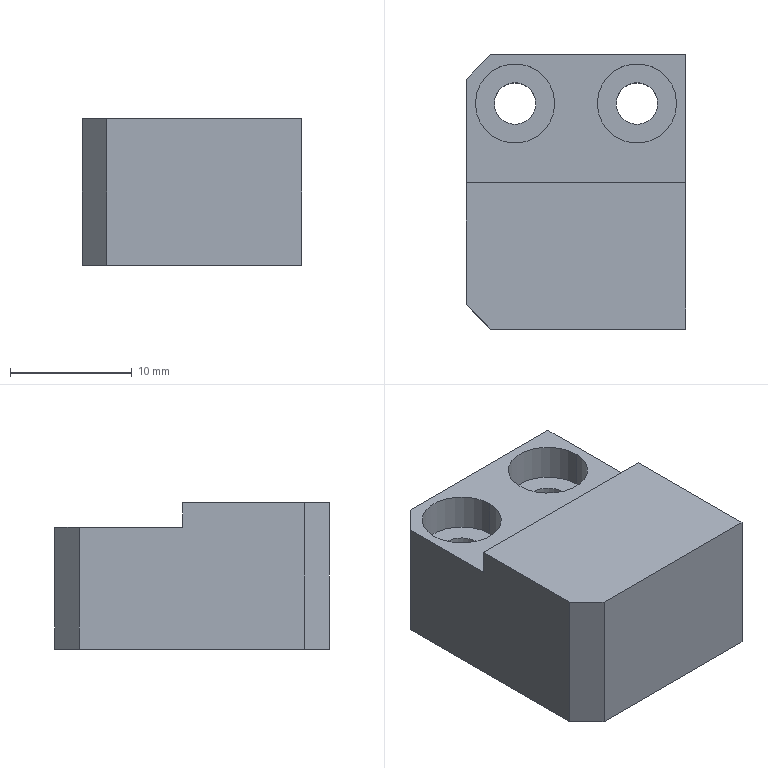Component | SolidWorks | ClampB-1 | 1 solid | 23 faces | box 18 x 22.5 x 12 mm | volume 3358 mm3 | plane 13 | cylinder 10 | commonest cylinder face diameters 6.5 x4 3.4 x4 8 x2
build123d program:
from build123d import *

# Parameters (mm, degrees)
SKETCH1_W                                            = 10
SKETCH1_H                                            = 22.5
EXTRUDE1_DEPTH                                       = 18
M3_HEX_SOCKET_HEAD_CAP_SCREW_COUNTERBORE_D           = 3.4
M3_HEX_SOCKET_HEAD_CAP_SCREW_COUNTERBORE_CBORE_D     = 6.5
M3_HEX_SOCKET_HEAD_CAP_SCREW_COUNTERBORE_CBORE_DEPTH = 3
SKETCH4_W                                            = 18
SKETCH4_H                                            = 12
EXTRUDE2_DEPTH                                       = 2
SKETCH5_R                                            = 4
EXTRUDE3_DEPTH                                       = 15
CHAMFER2_SIZE                                        = 2


with BuildPart() as part:
    # Sketch1 → Extrude1 (new body)
    with BuildSketch(Plane.XY):
        Rectangle(SKETCH1_W, SKETCH1_H)
    extrude(amount=EXTRUDE1_DEPTH)

    # M3 Hex Socket Head Cap Screw Counterbore (through all)
    with Locations(Plane(origin=(5, 0, 0), x_dir=(0, 0, -1), z_dir=(1, 0, 0))):
        with Locations((-4, 7.25), (-14, 7.25)):
            CounterBoreHole(M3_HEX_SOCKET_HEAD_CAP_SCREW_COUNTERBORE_D / 2, M3_HEX_SOCKET_HEAD_CAP_SCREW_COUNTERBORE_CBORE_D / 2, M3_HEX_SOCKET_HEAD_CAP_SCREW_COUNTERBORE_CBORE_DEPTH)

    # Sketch4 → Extrude2 (add)
    with BuildSketch(Plane(origin=(5, 0, 0), x_dir=(0, 0, -1), z_dir=(1, 0, 0))):
        with Locations((-9, -5.25)):
            Rectangle(SKETCH4_W, SKETCH4_H)
    extrude(amount=EXTRUDE2_DEPTH)

    # Sketch5 → Extrude3 (cut)
    with BuildSketch(Plane(origin=(0, 0, 0), x_dir=(-1, 0, 0), z_dir=(0, 0, -1))):
        with Locations((-2, -5.25)):
            Circle(SKETCH5_R)
    extrude(amount=-EXTRUDE3_DEPTH, mode=Mode.SUBTRACT)

    # Chamfer2
    chamfer2_edges = [part.edges().sort_by_distance(p)[0] for p in [
        (0, 11.25, 18),
        (1, -11.25, 18),
    ]]
    chamfer(chamfer2_edges, length=CHAMFER2_SIZE)


solid = part.part

# Placed as in the assembly
solid = solid.moved(Location((-68, 36.25, 15), (0, -90, 0)))
STEP:
#1=COLOUR_RGB('',0.7922,0.8196,0.9333);
#2=FILL_AREA_STYLE_COLOUR('',#1);
#3=FILL_AREA_STYLE('',(#2));
#4=SURFACE_STYLE_FILL_AREA(#3);
#5=SURFACE_SIDE_STYLE('',(#4));
#6=SURFACE_STYLE_USAGE(.BOTH.,#5);
#7=PRESENTATION_STYLE_ASSIGNMENT((#6));
#8=CARTESIAN_POINT('',(-3.268,1.22,0.8268));
#9=VERTEX_POINT('',#8);
#10=CARTESIAN_POINT('',(-3.268,1.22,0.5118));
#11=VERTEX_POINT('',#10);
#12=CARTESIAN_POINT('',(-3.268,1.22,0.6693));
#13=DIRECTION('',(1.,0.,0.));
#14=DIRECTION('',(0.,0.,-1.));
#15=AXIS2_PLACEMENT_3D('',#12,#13,#14);
#16=CIRCLE('',#15,0.1575);
#17=EDGE_CURVE('',#9,#11,#16,.T.);
#18=ORIENTED_EDGE('',*,*,#17,.F.);
#19=CARTESIAN_POINT('',(-2.677,1.22,0.8268));
#20=VERTEX_POINT('',#19);
#21=CARTESIAN_POINT('',(-3.268,1.22,0.8268));
#22=DIRECTION('',(1.,0.,0.));
#23=VECTOR('',#22,39.37);
#24=LINE('',#21,#23);
#25=EDGE_CURVE('',#9,#20,#24,.T.);
#26=ORIENTED_EDGE('',*,*,#25,.T.);
#27=CARTESIAN_POINT('',(-2.677,1.22,0.5118));
#28=VERTEX_POINT('',#27);
#29=CARTESIAN_POINT('',(-2.677,1.22,0.6693));
#30=DIRECTION('',(1.,0.,0.));
#31=DIRECTION('',(0.,0.,-1.));
#32=AXIS2_PLACEMENT_3D('',#29,#30,#31);
#33=CIRCLE('',#32,0.1575);
#34=EDGE_CURVE('',#20,#28,#33,.T.);
#35=ORIENTED_EDGE('',*,*,#34,.T.);
#36=CARTESIAN_POINT('',(-3.268,1.22,0.5118));
#37=DIRECTION('',(1.,0.,0.));
#38=VECTOR('',#37,39.37);
#39=LINE('',#36,#38);
#40=EDGE_CURVE('',#11,#28,#39,.T.);
#41=ORIENTED_EDGE('',*,*,#40,.F.);
#42=EDGE_LOOP('',(#18,#26,#35,#41));
#43=FACE_OUTER_BOUND('',#42,.T.);
#44=CARTESIAN_POINT('',(-3.268,1.22,0.6693));
#45=DIRECTION('',(1.,0.,0.));
#46=DIRECTION('',(0.,0.,-1.));
#47=AXIS2_PLACEMENT_3D('',#44,#45,#46);
#48=CYLINDRICAL_SURFACE('',#47,0.1575);
#49=ADVANCED_FACE('',(#43),#48,.F.);
#50=CARTESIAN_POINT('',(-2.963,1.713,0.6693));
#51=VERTEX_POINT('',#50);
#52=CARTESIAN_POINT('',(-2.707,1.713,0.6693));
#53=VERTEX_POINT('',#52);
#54=CARTESIAN_POINT('',(-2.835,1.713,0.6693));
#55=DIRECTION('',(0.,0.,1.));
#56=DIRECTION('',(1.,0.,0.));
#57=AXIS2_PLACEMENT_3D('',#54,#55,#56);
#58=CIRCLE('',#57,0.128);
#59=EDGE_CURVE('',#51,#53,#58,.T.);
#60=ORIENTED_EDGE('',*,*,#59,.F.);
#61=CARTESIAN_POINT('',(-2.963,1.713,0.7874));
#62=VERTEX_POINT('',#61);
#63=CARTESIAN_POINT('',(-2.963,1.713,0.7874));
#64=DIRECTION('',(0.,0.,1.));
#65=VECTOR('',#64,39.37);
#66=LINE('',#63,#65);
#67=EDGE_CURVE('',#51,#62,#66,.T.);
#68=ORIENTED_EDGE('',*,*,#67,.T.);
#69=CARTESIAN_POINT('',(-2.707,1.713,0.7874));
#70=VERTEX_POINT('',#69);
#71=CARTESIAN_POINT('',(-2.835,1.713,0.7874));
#72=DIRECTION('',(0.,0.,1.));
#73=DIRECTION('',(1.,0.,0.));
#74=AXIS2_PLACEMENT_3D('',#71,#72,#73);
#75=CIRCLE('',#74,0.128);
#76=EDGE_CURVE('',#62,#70,#75,.T.);
#77=ORIENTED_EDGE('',*,*,#76,.T.);
#78=CARTESIAN_POINT('',(-2.707,1.713,0.7874));
#79=DIRECTION('',(0.,0.,1.));
#80=VECTOR('',#79,39.37);
#81=LINE('',#78,#80);
#82=EDGE_CURVE('',#53,#70,#81,.T.);
#83=ORIENTED_EDGE('',*,*,#82,.F.);
#84=EDGE_LOOP('',(#60,#68,#77,#83));
#85=FACE_OUTER_BOUND('',#84,.T.);
#86=CARTESIAN_POINT('',(-2.835,1.713,0.7874));
#87=DIRECTION('',(0.,0.,1.));
#88=DIRECTION('',(1.,0.,0.));
#89=AXIS2_PLACEMENT_3D('',#86,#87,#88);
#90=CYLINDRICAL_SURFACE('',#89,0.128);
#91=ADVANCED_FACE('',(#85),#90,.F.);
#92=CARTESIAN_POINT('',(-2.902,1.713,0.3937));
#93=VERTEX_POINT('',#92);
#94=CARTESIAN_POINT('',(-2.768,1.713,0.3937));
#95=VERTEX_POINT('',#94);
#96=CARTESIAN_POINT('',(-2.835,1.713,0.3937));
#97=DIRECTION('',(0.,0.,1.));
#98=DIRECTION('',(1.,0.,0.));
#99=AXIS2_PLACEMENT_3D('',#96,#97,#98);
#100=CIRCLE('',#99,0.06693);
#101=EDGE_CURVE('',#93,#95,#100,.T.);
#102=ORIENTED_EDGE('',*,*,#101,.F.);
#103=CARTESIAN_POINT('',(-2.902,1.713,0.6693));
#104=VERTEX_POINT('',#103);
#105=CARTESIAN_POINT('',(-2.902,1.713,0.7874));
#106=DIRECTION('',(0.,0.,1.));
#107=VECTOR('',#106,39.37);
#108=LINE('',#105,#107);
#109=EDGE_CURVE('',#93,#104,#108,.T.);
#110=ORIENTED_EDGE('',*,*,#109,.T.);
#111=CARTESIAN_POINT('',(-2.768,1.713,0.6693));
#112=VERTEX_POINT('',#111);
#113=CARTESIAN_POINT('',(-2.835,1.713,0.6693));
#114=DIRECTION('',(0.,0.,1.));
#115=DIRECTION('',(1.,0.,0.));
#116=AXIS2_PLACEMENT_3D('',#113,#114,#115);
#117=CIRCLE('',#116,0.06693);
#118=EDGE_CURVE('',#104,#112,#117,.T.);
#119=ORIENTED_EDGE('',*,*,#118,.T.);
#120=CARTESIAN_POINT('',(-2.768,1.713,0.7874));
#121=DIRECTION('',(0.,0.,1.));
#122=VECTOR('',#121,39.37);
#123=LINE('',#120,#122);
#124=EDGE_CURVE('',#95,#112,#123,.T.);
#125=ORIENTED_EDGE('',*,*,#124,.F.);
#126=EDGE_LOOP('',(#102,#110,#119,#125));
#127=FACE_OUTER_BOUND('',#126,.T.);
#128=CARTESIAN_POINT('',(-2.835,1.713,0.7874));
#129=DIRECTION('',(0.,0.,1.));
#130=DIRECTION('',(1.,0.,0.));
#131=AXIS2_PLACEMENT_3D('',#128,#129,#130);
#132=CYLINDRICAL_SURFACE('',#131,0.06693);
#133=ADVANCED_FACE('',(#127),#132,.F.);
#134=CARTESIAN_POINT('',(-3.356,1.713,0.6693));
#135=VERTEX_POINT('',#134);
#136=CARTESIAN_POINT('',(-3.1,1.713,0.6693));
#137=VERTEX_POINT('',#136);
#138=CARTESIAN_POINT('',(-3.228,1.713,0.6693));
#139=DIRECTION('',(0.,0.,1.));
#140=DIRECTION('',(1.,0.,0.));
#141=AXIS2_PLACEMENT_3D('',#138,#139,#140);
#142=CIRCLE('',#141,0.128);
#143=EDGE_CURVE('',#135,#137,#142,.T.);
#144=ORIENTED_EDGE('',*,*,#143,.F.);
#145=CARTESIAN_POINT('',(-3.356,1.713,0.7874));
#146=VERTEX_POINT('',#145);
#147=CARTESIAN_POINT('',(-3.356,1.713,0.7874));
#148=DIRECTION('',(0.,0.,1.));
#149=VECTOR('',#148,39.37);
#150=LINE('',#147,#149);
#151=EDGE_CURVE('',#135,#146,#150,.T.);
#152=ORIENTED_EDGE('',*,*,#151,.T.);
#153=CARTESIAN_POINT('',(-3.1,1.713,0.7874));
#154=VERTEX_POINT('',#153);
#155=CARTESIAN_POINT('',(-3.228,1.713,0.7874));
#156=DIRECTION('',(0.,0.,1.));
#157=DIRECTION('',(1.,0.,0.));
#158=AXIS2_PLACEMENT_3D('',#155,#156,#157);
#159=CIRCLE('',#158,0.128);
#160=EDGE_CURVE('',#146,#154,#159,.T.);
#161=ORIENTED_EDGE('',*,*,#160,.T.);
#162=CARTESIAN_POINT('',(-3.1,1.713,0.7874));
#163=DIRECTION('',(0.,0.,1.));
#164=VECTOR('',#163,39.37);
#165=LINE('',#162,#164);
#166=EDGE_CURVE('',#137,#154,#165,.T.);
#167=ORIENTED_EDGE('',*,*,#166,.F.);
#168=EDGE_LOOP('',(#144,#152,#161,#167));
#169=FACE_OUTER_BOUND('',#168,.T.);
#170=CARTESIAN_POINT('',(-3.228,1.713,0.7874));
#171=DIRECTION('',(0.,0.,1.));
#172=DIRECTION('',(1.,0.,0.));
#173=AXIS2_PLACEMENT_3D('',#170,#171,#172);
#174=CYLINDRICAL_SURFACE('',#173,0.128);
#175=ADVANCED_FACE('',(#169),#174,.F.);
#176=CARTESIAN_POINT('',(-3.295,1.713,0.3937));
#177=VERTEX_POINT('',#176);
#178=CARTESIAN_POINT('',(-3.161,1.713,0.3937));
#179=VERTEX_POINT('',#178);
#180=CARTESIAN_POINT('',(-3.228,1.713,0.3937));
#181=DIRECTION('',(0.,0.,1.));
#182=DIRECTION('',(1.,0.,0.));
#183=AXIS2_PLACEMENT_3D('',#180,#181,#182);
#184=CIRCLE('',#183,0.06693);
#185=EDGE_CURVE('',#177,#179,#184,.T.);
#186=ORIENTED_EDGE('',*,*,#185,.F.);
#187=CARTESIAN_POINT('',(-3.295,1.713,0.6693));
#188=VERTEX_POINT('',#187);
#189=CARTESIAN_POINT('',(-3.295,1.713,0.7874));
#190=DIRECTION('',(0.,0.,1.));
#191=VECTOR('',#190,39.37);
#192=LINE('',#189,#191);
#193=EDGE_CURVE('',#177,#188,#192,.T.);
#194=ORIENTED_EDGE('',*,*,#193,.T.);
#195=CARTESIAN_POINT('',(-3.161,1.713,0.6693));
#196=VERTEX_POINT('',#195);
#197=CARTESIAN_POINT('',(-3.228,1.713,0.6693));
#198=DIRECTION('',(0.,0.,1.));
#199=DIRECTION('',(1.,0.,0.));
#200=AXIS2_PLACEMENT_3D('',#197,#198,#199);
#201=CIRCLE('',#200,0.06693);
#202=EDGE_CURVE('',#188,#196,#201,.T.);
#203=ORIENTED_EDGE('',*,*,#202,.T.);
#204=CARTESIAN_POINT('',(-3.161,1.713,0.7874));
#205=DIRECTION('',(0.,0.,1.));
#206=VECTOR('',#205,39.37);
#207=LINE('',#204,#206);
#208=EDGE_CURVE('',#179,#196,#207,.T.);
#209=ORIENTED_EDGE('',*,*,#208,.F.);
#210=EDGE_LOOP('',(#186,#194,#203,#209));
#211=FACE_OUTER_BOUND('',#210,.T.);
#212=CARTESIAN_POINT('',(-3.228,1.713,0.7874));
#213=DIRECTION('',(0.,0.,1.));
#214=DIRECTION('',(1.,0.,0.));
#215=AXIS2_PLACEMENT_3D('',#212,#213,#214);
#216=CYLINDRICAL_SURFACE('',#215,0.06693);
#217=ADVANCED_FACE('',(#211),#216,.F.);
#218=CARTESIAN_POINT('',(-3.228,1.713,0.7874));
#219=DIRECTION('',(0.,0.,1.));
#220=DIRECTION('',(1.,0.,0.));
#221=AXIS2_PLACEMENT_3D('',#218,#219,#220);
#222=CIRCLE('',#221,0.128);
#223=EDGE_CURVE('',#154,#146,#222,.T.);
#224=ORIENTED_EDGE('',*,*,#223,.F.);
#225=ORIENTED_EDGE('',*,*,#160,.F.);
#226=EDGE_LOOP('',(#224,#225));
#227=FACE_BOUND('',#226,.T.);
#228=CARTESIAN_POINT('',(-2.835,1.713,0.7874));
#229=DIRECTION('',(0.,0.,1.));
#230=DIRECTION('',(1.,0.,0.));
#231=AXIS2_PLACEMENT_3D('',#228,#229,#230);
#232=CIRCLE('',#231,0.128);
#233=EDGE_CURVE('',#70,#62,#232,.T.);
#234=ORIENTED_EDGE('',*,*,#233,.F.);
#235=ORIENTED_EDGE('',*,*,#76,.F.);
#236=EDGE_LOOP('',(#234,#235));
#237=FACE_BOUND('',#236,.T.);
#238=CARTESIAN_POINT('',(-3.307,1.87,0.7874));
#239=VERTEX_POINT('',#238);
#240=CARTESIAN_POINT('',(-2.677,1.87,0.7874));
#241=VERTEX_POINT('',#240);
#242=CARTESIAN_POINT('',(-3.386,1.87,0.7874));
#243=DIRECTION('',(1.,0.,0.));
#244=VECTOR('',#243,39.37);
#245=LINE('',#242,#244);
#246=EDGE_CURVE('',#239,#241,#245,.T.);
#247=ORIENTED_EDGE('',*,*,#246,.F.);
#248=CARTESIAN_POINT('',(-3.386,1.791,0.7874));
#249=VERTEX_POINT('',#248);
#250=CARTESIAN_POINT('',(-3.386,1.791,0.7874));
#251=DIRECTION('',(-0.7071,-0.7071,0.));
#252=VECTOR('',#251,39.37);
#253=LINE('',#250,#252);
#254=EDGE_CURVE('',#239,#249,#253,.T.);
#255=ORIENTED_EDGE('',*,*,#254,.T.);
#256=CARTESIAN_POINT('',(-3.386,1.457,0.7874));
#257=VERTEX_POINT('',#256);
#258=CARTESIAN_POINT('',(-3.386,0.9843,0.7874));
#259=DIRECTION('',(0.,1.,0.));
#260=VECTOR('',#259,39.37);
#261=LINE('',#258,#260);
#262=EDGE_CURVE('',#257,#249,#261,.T.);
#263=ORIENTED_EDGE('',*,*,#262,.F.);
#264=CARTESIAN_POINT('',(-2.677,1.457,0.7874));
#265=VERTEX_POINT('',#264);
#266=CARTESIAN_POINT('',(-3.386,1.457,0.7874));
#267=DIRECTION('',(-1.,0.,0.));
#268=VECTOR('',#267,39.37);
#269=LINE('',#266,#268);
#270=EDGE_CURVE('',#265,#257,#269,.T.);
#271=ORIENTED_EDGE('',*,*,#270,.F.);
#272=CARTESIAN_POINT('',(-2.677,0.9843,0.7874));
#273=DIRECTION('',(0.,1.,0.));
#274=VECTOR('',#273,39.37);
#275=LINE('',#272,#274);
#276=EDGE_CURVE('',#265,#241,#275,.T.);
#277=ORIENTED_EDGE('',*,*,#276,.T.);
#278=EDGE_LOOP('',(#247,#255,#263,#271,#277));
#279=FACE_OUTER_BOUND('',#278,.T.);
#280=CARTESIAN_POINT('',(-3.386,0.9843,0.7874));
#281=DIRECTION('',(0.,0.,-1.));
#282=DIRECTION('',(-1.,0.,0.));
#283=AXIS2_PLACEMENT_3D('',#280,#281,#282);
#284=PLANE('',#283);
#285=ADVANCED_FACE('',(#227,#237,#279),#284,.F.);
#286=CARTESIAN_POINT('',(-2.835,1.713,0.3937));
#287=DIRECTION('',(0.,0.,1.));
#288=DIRECTION('',(1.,0.,0.));
#289=AXIS2_PLACEMENT_3D('',#286,#287,#288);
#290=CIRCLE('',#289,0.06693);
#291=EDGE_CURVE('',#95,#93,#290,.T.);
#292=ORIENTED_EDGE('',*,*,#291,.T.);
#293=ORIENTED_EDGE('',*,*,#101,.T.);
#294=EDGE_LOOP('',(#292,#293));
#295=FACE_BOUND('',#294,.T.);
#296=CARTESIAN_POINT('',(-3.228,1.713,0.3937));
#297=DIRECTION('',(0.,0.,1.));
#298=DIRECTION('',(1.,0.,0.));
#299=AXIS2_PLACEMENT_3D('',#296,#297,#298);
#300=CIRCLE('',#299,0.06693);
#301=EDGE_CURVE('',#179,#177,#300,.T.);
#302=ORIENTED_EDGE('',*,*,#301,.T.);
#303=ORIENTED_EDGE('',*,*,#185,.T.);
#304=EDGE_LOOP('',(#302,#303));
#305=FACE_BOUND('',#304,.T.);
#306=CARTESIAN_POINT('',(-3.386,1.791,0.3937));
#307=VERTEX_POINT('',#306);
#308=CARTESIAN_POINT('',(-3.386,1.063,0.3937));
#309=VERTEX_POINT('',#308);
#310=CARTESIAN_POINT('',(-3.386,0.9843,0.3937));
#311=DIRECTION('',(0.,-1.,0.));
#312=VECTOR('',#311,39.37);
#313=LINE('',#310,#312);
#314=EDGE_CURVE('',#307,#309,#313,.T.);
#315=ORIENTED_EDGE('',*,*,#314,.F.);
#316=CARTESIAN_POINT('',(-3.307,1.87,0.3937));
#317=VERTEX_POINT('',#316);
#318=CARTESIAN_POINT('',(-3.386,1.791,0.3937));
#319=DIRECTION('',(0.7071,0.7071,0.));
#320=VECTOR('',#319,39.37);
#321=LINE('',#318,#320);
#322=EDGE_CURVE('',#307,#317,#321,.T.);
#323=ORIENTED_EDGE('',*,*,#322,.T.);
#324=CARTESIAN_POINT('',(-2.677,1.87,0.3937));
#325=VERTEX_POINT('',#324);
#326=CARTESIAN_POINT('',(-3.386,1.87,0.3937));
#327=DIRECTION('',(1.,0.,0.));
#328=VECTOR('',#327,39.37);
#329=LINE('',#326,#328);
#330=EDGE_CURVE('',#317,#325,#329,.T.);
#331=ORIENTED_EDGE('',*,*,#330,.T.);
#332=CARTESIAN_POINT('',(-2.677,0.9843,0.3937));
#333=VERTEX_POINT('',#332);
#334=CARTESIAN_POINT('',(-2.677,0.9843,0.3937));
#335=DIRECTION('',(0.,-1.,0.));
#336=VECTOR('',#335,39.37);
#337=LINE('',#334,#336);
#338=EDGE_CURVE('',#325,#333,#337,.T.);
#339=ORIENTED_EDGE('',*,*,#338,.T.);
#340=CARTESIAN_POINT('',(-3.307,0.9843,0.3937));
#341=VERTEX_POINT('',#340);
#342=CARTESIAN_POINT('',(-3.386,0.9843,0.3937));
#343=DIRECTION('',(1.,0.,0.));
#344=VECTOR('',#343,39.37);
#345=LINE('',#342,#344);
#346=EDGE_CURVE('',#341,#333,#345,.T.);
#347=ORIENTED_EDGE('',*,*,#346,.F.);
#348=CARTESIAN_POINT('',(-3.386,1.063,0.3937));
#349=DIRECTION('',(-0.7071,0.7071,0.));
#350=VECTOR('',#349,39.37);
#351=LINE('',#348,#350);
#352=EDGE_CURVE('',#341,#309,#351,.T.);
#353=ORIENTED_EDGE('',*,*,#352,.T.);
#354=EDGE_LOOP('',(#315,#323,#331,#339,#347,#353));
#355=FACE_OUTER_BOUND('',#354,.T.);
#356=CARTESIAN_POINT('',(-3.386,0.9843,0.3937));
#357=DIRECTION('',(0.,0.,1.));
#358=DIRECTION('',(1.,0.,0.));
#359=AXIS2_PLACEMENT_3D('',#356,#357,#358);
#360=PLANE('',#359);
#361=ADVANCED_FACE('',(#295,#305,#355),#360,.F.);
#362=CARTESIAN_POINT('',(-3.307,0.9843,0.8661));
#363=VERTEX_POINT('',#362);
#364=CARTESIAN_POINT('',(-2.677,0.9843,0.8661));
#365=VERTEX_POINT('',#364);
#366=CARTESIAN_POINT('',(-3.386,0.9843,0.8661));
#367=DIRECTION('',(1.,0.,0.));
#368=VECTOR('',#367,39.37);
#369=LINE('',#366,#368);
#370=EDGE_CURVE('',#363,#365,#369,.T.);
#371=ORIENTED_EDGE('',*,*,#370,.F.);
#372=CARTESIAN_POINT('',(-3.307,0.9843,0.3937));
#373=DIRECTION('',(0.,0.,-1.));
#374=VECTOR('',#373,39.37);
#375=LINE('',#372,#374);
#376=EDGE_CURVE('',#363,#341,#375,.T.);
#377=ORIENTED_EDGE('',*,*,#376,.T.);
#378=ORIENTED_EDGE('',*,*,#346,.T.);
#379=CARTESIAN_POINT('',(-2.677,0.9843,0.7874));
#380=DIRECTION('',(0.,0.,1.));
#381=VECTOR('',#380,39.37);
#382=LINE('',#379,#381);
#383=EDGE_CURVE('',#333,#365,#382,.T.);
#384=ORIENTED_EDGE('',*,*,#383,.T.);
#385=EDGE_LOOP('',(#371,#377,#378,#384));
#386=FACE_OUTER_BOUND('',#385,.T.);
#387=CARTESIAN_POINT('',(-3.386,0.9843,0.7874));
#388=DIRECTION('',(0.,1.,0.));
#389=DIRECTION('',(-1.,0.,0.));
#390=AXIS2_PLACEMENT_3D('',#387,#388,#389);
#391=PLANE('',#390);
#392=ADVANCED_FACE('',(#386),#391,.F.);
#393=ORIENTED_EDGE('',*,*,#330,.F.);
#394=CARTESIAN_POINT('',(-3.307,1.87,0.7874));
#395=DIRECTION('',(0.,0.,1.));
#396=VECTOR('',#395,39.37);
#397=LINE('',#394,#396);
#398=EDGE_CURVE('',#317,#239,#397,.T.);
#399=ORIENTED_EDGE('',*,*,#398,.T.);
#400=ORIENTED_EDGE('',*,*,#246,.T.);
#401=CARTESIAN_POINT('',(-2.677,1.87,0.7874));
#402=DIRECTION('',(0.,-0.,-1.));
#403=VECTOR('',#402,39.37);
#404=LINE('',#401,#403);
#405=EDGE_CURVE('',#241,#325,#404,.T.);
#406=ORIENTED_EDGE('',*,*,#405,.T.);
#407=EDGE_LOOP('',(#393,#399,#400,#406));
#408=FACE_OUTER_BOUND('',#407,.T.);
#409=CARTESIAN_POINT('',(-3.386,1.87,0.7874));
#410=DIRECTION('',(0.,-1.,0.));
#411=DIRECTION('',(0.,0.,1.));
#412=AXIS2_PLACEMENT_3D('',#409,#410,#411);
#413=PLANE('',#412);
#414=ADVANCED_FACE('',(#408),#413,.F.);
#415=ORIENTED_EDGE('',*,*,#262,.T.);
#416=CARTESIAN_POINT('',(-3.386,1.791,0.3937));
#417=DIRECTION('',(0.,-0.,-1.));
#418=VECTOR('',#417,39.37);
#419=LINE('',#416,#418);
#420=EDGE_CURVE('',#249,#307,#419,.T.);
#421=ORIENTED_EDGE('',*,*,#420,.T.);
#422=ORIENTED_EDGE('',*,*,#314,.T.);
#423=CARTESIAN_POINT('',(-3.386,1.063,0.8661));
#424=VERTEX_POINT('',#423);
#425=CARTESIAN_POINT('',(-3.386,1.063,0.8661));
#426=DIRECTION('',(0.,0.,1.));
#427=VECTOR('',#426,39.37);
#428=LINE('',#425,#427);
#429=EDGE_CURVE('',#309,#424,#428,.T.);
#430=ORIENTED_EDGE('',*,*,#429,.T.);
#431=CARTESIAN_POINT('',(-3.386,1.457,0.8661));
#432=VERTEX_POINT('',#431);
#433=CARTESIAN_POINT('',(-3.386,0.9843,0.8661));
#434=DIRECTION('',(0.,-1.,0.));
#435=VECTOR('',#434,39.37);
#436=LINE('',#433,#435);
#437=EDGE_CURVE('',#432,#424,#436,.T.);
#438=ORIENTED_EDGE('',*,*,#437,.F.);
#439=CARTESIAN_POINT('',(-3.386,1.457,0.8661));
#440=DIRECTION('',(0.,0.,-1.));
#441=VECTOR('',#440,39.37);
#442=LINE('',#439,#441);
#443=EDGE_CURVE('',#432,#257,#442,.T.);
#444=ORIENTED_EDGE('',*,*,#443,.T.);
#445=EDGE_LOOP('',(#415,#421,#422,#430,#438,#444));
#446=FACE_OUTER_BOUND('',#445,.T.);
#447=CARTESIAN_POINT('',(-3.386,1.87,0.3937));
#448=DIRECTION('',(-1.,0.,0.));
#449=DIRECTION('',(0.,0.,1.));
#450=AXIS2_PLACEMENT_3D('',#447,#448,#449);
#451=PLANE('',#450);
#452=ADVANCED_FACE('',(#446),#451,.T.);
#453=CARTESIAN_POINT('',(-2.677,1.22,0.6693));
#454=DIRECTION('',(1.,0.,0.));
#455=DIRECTION('',(0.,0.,-1.));
#456=AXIS2_PLACEMENT_3D('',#453,#454,#455);
#457=CIRCLE('',#456,0.1575);
#458=EDGE_CURVE('',#28,#20,#457,.T.);
#459=ORIENTED_EDGE('',*,*,#458,.F.);
#460=ORIENTED_EDGE('',*,*,#34,.F.);
#461=EDGE_LOOP('',(#459,#460));
#462=FACE_BOUND('',#461,.T.);
#463=ORIENTED_EDGE('',*,*,#338,.F.);
#464=ORIENTED_EDGE('',*,*,#405,.F.);
#465=ORIENTED_EDGE('',*,*,#276,.F.);
#466=CARTESIAN_POINT('',(-2.677,1.457,0.8661));
#467=VERTEX_POINT('',#466);
#468=CARTESIAN_POINT('',(-2.677,1.457,0.8661));
#469=DIRECTION('',(0.,0.,-1.));
#470=VECTOR('',#469,39.37);
#471=LINE('',#468,#470);
#472=EDGE_CURVE('',#467,#265,#471,.T.);
#473=ORIENTED_EDGE('',*,*,#472,.F.);
#474=CARTESIAN_POINT('',(-2.677,0.9843,0.8661));
#475=DIRECTION('',(0.,1.,0.));
#476=VECTOR('',#475,39.37);
#477=LINE('',#474,#476);
#478=EDGE_CURVE('',#365,#467,#477,.T.);
#479=ORIENTED_EDGE('',*,*,#478,.F.);
#480=ORIENTED_EDGE('',*,*,#383,.F.);
#481=EDGE_LOOP('',(#463,#464,#465,#473,#479,#480));
#482=FACE_OUTER_BOUND('',#481,.T.);
#483=CARTESIAN_POINT('',(-2.677,1.87,0.3937));
#484=DIRECTION('',(-1.,0.,0.));
#485=DIRECTION('',(0.,0.,1.));
#486=AXIS2_PLACEMENT_3D('',#483,#484,#485);
#487=PLANE('',#486);
#488=ADVANCED_FACE('',(#462,#482),#487,.F.);
#489=ORIENTED_EDGE('',*,*,#193,.F.);
#490=ORIENTED_EDGE('',*,*,#301,.F.);
#491=ORIENTED_EDGE('',*,*,#208,.T.);
#492=CARTESIAN_POINT('',(-3.228,1.713,0.6693));
#493=DIRECTION('',(0.,0.,1.));
#494=DIRECTION('',(1.,0.,0.));
#495=AXIS2_PLACEMENT_3D('',#492,#493,#494);
#496=CIRCLE('',#495,0.06693);
#497=EDGE_CURVE('',#196,#188,#496,.T.);
#498=ORIENTED_EDGE('',*,*,#497,.T.);
#499=EDGE_LOOP('',(#489,#490,#491,#498));
#500=FACE_OUTER_BOUND('',#499,.T.);
#501=CARTESIAN_POINT('',(-3.228,1.713,0.7874));
#502=DIRECTION('',(0.,0.,1.));
#503=DIRECTION('',(1.,0.,0.));
#504=AXIS2_PLACEMENT_3D('',#501,#502,#503);
#505=CYLINDRICAL_SURFACE('',#504,0.06693);
#506=ADVANCED_FACE('',(#500),#505,.F.);
#507=ORIENTED_EDGE('',*,*,#497,.F.);
#508=ORIENTED_EDGE('',*,*,#202,.F.);
#509=EDGE_LOOP('',(#507,#508));
#510=FACE_BOUND('',#509,.T.);
#511=CARTESIAN_POINT('',(-3.228,1.713,0.6693));
#512=DIRECTION('',(0.,0.,1.));
#513=DIRECTION('',(1.,0.,0.));
#514=AXIS2_PLACEMENT_3D('',#511,#512,#513);
#515=CIRCLE('',#514,0.128);
#516=EDGE_CURVE('',#137,#135,#515,.T.);
#517=ORIENTED_EDGE('',*,*,#516,.T.);
#518=ORIENTED_EDGE('',*,*,#143,.T.);
#519=EDGE_LOOP('',(#517,#518));
#520=FACE_OUTER_BOUND('',#519,.T.);
#521=CARTESIAN_POINT('',(-3.228,1.78,0.6693));
#522=DIRECTION('',(0.,0.,-1.));
#523=DIRECTION('',(-1.,0.,0.));
#524=AXIS2_PLACEMENT_3D('',#521,#522,#523);
#525=PLANE('',#524);
#526=ADVANCED_FACE('',(#510,#520),#525,.F.);
#527=ORIENTED_EDGE('',*,*,#151,.F.);
#528=ORIENTED_EDGE('',*,*,#516,.F.);
#529=ORIENTED_EDGE('',*,*,#166,.T.);
#530=ORIENTED_EDGE('',*,*,#223,.T.);
#531=EDGE_LOOP('',(#527,#528,#529,#530));
#532=FACE_OUTER_BOUND('',#531,.T.);
#533=CARTESIAN_POINT('',(-3.228,1.713,0.7874));
#534=DIRECTION('',(0.,0.,1.));
#535=DIRECTION('',(1.,0.,0.));
#536=AXIS2_PLACEMENT_3D('',#533,#534,#535);
#537=CYLINDRICAL_SURFACE('',#536,0.128);
#538=ADVANCED_FACE('',(#532),#537,.F.);
#539=ORIENTED_EDGE('',*,*,#109,.F.);
#540=ORIENTED_EDGE('',*,*,#291,.F.);
#541=ORIENTED_EDGE('',*,*,#124,.T.);
#542=CARTESIAN_POINT('',(-2.835,1.713,0.6693));
#543=DIRECTION('',(0.,0.,1.));
#544=DIRECTION('',(1.,0.,0.));
#545=AXIS2_PLACEMENT_3D('',#542,#543,#544);
#546=CIRCLE('',#545,0.06693);
#547=EDGE_CURVE('',#112,#104,#546,.T.);
#548=ORIENTED_EDGE('',*,*,#547,.T.);
#549=EDGE_LOOP('',(#539,#540,#541,#548));
#550=FACE_OUTER_BOUND('',#549,.T.);
#551=CARTESIAN_POINT('',(-2.835,1.713,0.7874));
#552=DIRECTION('',(0.,0.,1.));
#553=DIRECTION('',(1.,0.,0.));
#554=AXIS2_PLACEMENT_3D('',#551,#552,#553);
#555=CYLINDRICAL_SURFACE('',#554,0.06693);
#556=ADVANCED_FACE('',(#550),#555,.F.);
#557=ORIENTED_EDGE('',*,*,#547,.F.);
#558=ORIENTED_EDGE('',*,*,#118,.F.);
#559=EDGE_LOOP('',(#557,#558));
#560=FACE_BOUND('',#559,.T.);
#561=CARTESIAN_POINT('',(-2.835,1.713,0.6693));
#562=DIRECTION('',(0.,0.,1.));
#563=DIRECTION('',(1.,0.,0.));
#564=AXIS2_PLACEMENT_3D('',#561,#562,#563);
#565=CIRCLE('',#564,0.128);
#566=EDGE_CURVE('',#53,#51,#565,.T.);
#567=ORIENTED_EDGE('',*,*,#566,.T.);
#568=ORIENTED_EDGE('',*,*,#59,.T.);
#569=EDGE_LOOP('',(#567,#568));
#570=FACE_OUTER_BOUND('',#569,.T.);
#571=CARTESIAN_POINT('',(-2.835,1.78,0.6693));
#572=DIRECTION('',(0.,0.,-1.));
#573=DIRECTION('',(-1.,0.,0.));
#574=AXIS2_PLACEMENT_3D('',#571,#572,#573);
#575=PLANE('',#574);
#576=ADVANCED_FACE('',(#560,#570),#575,.F.);
#577=ORIENTED_EDGE('',*,*,#67,.F.);
#578=ORIENTED_EDGE('',*,*,#566,.F.);
#579=ORIENTED_EDGE('',*,*,#82,.T.);
#580=ORIENTED_EDGE('',*,*,#233,.T.);
#581=EDGE_LOOP('',(#577,#578,#579,#580));
#582=FACE_OUTER_BOUND('',#581,.T.);
#583=CARTESIAN_POINT('',(-2.835,1.713,0.7874));
#584=DIRECTION('',(0.,0.,1.));
#585=DIRECTION('',(1.,0.,0.));
#586=AXIS2_PLACEMENT_3D('',#583,#584,#585);
#587=CYLINDRICAL_SURFACE('',#586,0.128);
#588=ADVANCED_FACE('',(#582),#587,.F.);
#589=ORIENTED_EDGE('',*,*,#270,.T.);
#590=ORIENTED_EDGE('',*,*,#443,.F.);
#591=CARTESIAN_POINT('',(-3.386,1.457,0.8661));
#592=DIRECTION('',(-1.,0.,0.));
#593=VECTOR('',#592,39.37);
#594=LINE('',#591,#593);
#595=EDGE_CURVE('',#467,#432,#594,.T.);
#596=ORIENTED_EDGE('',*,*,#595,.F.);
#597=ORIENTED_EDGE('',*,*,#472,.T.);
#598=EDGE_LOOP('',(#589,#590,#596,#597));
#599=FACE_OUTER_BOUND('',#598,.T.);
#600=CARTESIAN_POINT('',(-3.386,1.457,0.8661));
#601=DIRECTION('',(0.,-1.,0.));
#602=DIRECTION('',(1.,0.,0.));
#603=AXIS2_PLACEMENT_3D('',#600,#601,#602);
#604=PLANE('',#603);
#605=ADVANCED_FACE('',(#599),#604,.F.);
#606=ORIENTED_EDGE('',*,*,#437,.T.);
#607=CARTESIAN_POINT('',(-3.386,1.063,0.8661));
#608=DIRECTION('',(0.7071,-0.7071,0.));
#609=VECTOR('',#608,39.37);
#610=LINE('',#607,#609);
#611=EDGE_CURVE('',#424,#363,#610,.T.);
#612=ORIENTED_EDGE('',*,*,#611,.T.);
#613=ORIENTED_EDGE('',*,*,#370,.T.);
#614=ORIENTED_EDGE('',*,*,#478,.T.);
#615=ORIENTED_EDGE('',*,*,#595,.T.);
#616=EDGE_LOOP('',(#606,#612,#613,#614,#615));
#617=FACE_OUTER_BOUND('',#616,.T.);
#618=CARTESIAN_POINT('',(-3.386,1.457,0.8661));
#619=DIRECTION('',(0.,0.,-1.));
#620=DIRECTION('',(-1.,0.,0.));
#621=AXIS2_PLACEMENT_3D('',#618,#619,#620);
#622=PLANE('',#621);
#623=ADVANCED_FACE('',(#617),#622,.F.);
#624=ORIENTED_EDGE('',*,*,#25,.F.);
#625=CARTESIAN_POINT('',(-3.268,1.22,0.6693));
#626=DIRECTION('',(1.,0.,0.));
#627=DIRECTION('',(0.,0.,-1.));
#628=AXIS2_PLACEMENT_3D('',#625,#626,#627);
#629=CIRCLE('',#628,0.1575);
#630=EDGE_CURVE('',#11,#9,#629,.T.);
#631=ORIENTED_EDGE('',*,*,#630,.F.);
#632=ORIENTED_EDGE('',*,*,#40,.T.);
#633=ORIENTED_EDGE('',*,*,#458,.T.);
#634=EDGE_LOOP('',(#624,#631,#632,#633));
#635=FACE_OUTER_BOUND('',#634,.T.);
#636=CARTESIAN_POINT('',(-3.268,1.22,0.6693));
#637=DIRECTION('',(1.,0.,0.));
#638=DIRECTION('',(0.,0.,-1.));
#639=AXIS2_PLACEMENT_3D('',#636,#637,#638);
#640=CYLINDRICAL_SURFACE('',#639,0.1575);
#641=ADVANCED_FACE('',(#635),#640,.F.);
#642=ORIENTED_EDGE('',*,*,#630,.T.);
#643=ORIENTED_EDGE('',*,*,#17,.T.);
#644=EDGE_LOOP('',(#642,#643));
#645=FACE_OUTER_BOUND('',#644,.T.);
#646=CARTESIAN_POINT('',(-3.268,1.22,0.6693));
#647=DIRECTION('',(1.,0.,0.));
#648=DIRECTION('',(0.,0.,-1.));
#649=AXIS2_PLACEMENT_3D('',#646,#647,#648);
#650=PLANE('',#649);
#651=ADVANCED_FACE('',(#645),#650,.T.);
#652=ORIENTED_EDGE('',*,*,#254,.F.);
#653=ORIENTED_EDGE('',*,*,#398,.F.);
#654=ORIENTED_EDGE('',*,*,#322,.F.);
#655=ORIENTED_EDGE('',*,*,#420,.F.);
#656=EDGE_LOOP('',(#652,#653,#654,#655));
#657=FACE_OUTER_BOUND('',#656,.T.);
#658=CARTESIAN_POINT('',(-3.386,1.791,0.3937));
#659=DIRECTION('',(-0.7071,0.7071,-0.));
#660=DIRECTION('',(-0.7071,-0.7071,0.));
#661=AXIS2_PLACEMENT_3D('',#658,#659,#660);
#662=PLANE('',#661);
#663=ADVANCED_FACE('',(#657),#662,.T.);
#664=ORIENTED_EDGE('',*,*,#352,.F.);
#665=ORIENTED_EDGE('',*,*,#376,.F.);
#666=ORIENTED_EDGE('',*,*,#611,.F.);
#667=ORIENTED_EDGE('',*,*,#429,.F.);
#668=EDGE_LOOP('',(#664,#665,#666,#667));
#669=FACE_OUTER_BOUND('',#668,.T.);
#670=CARTESIAN_POINT('',(-3.386,1.063,0.3937));
#671=DIRECTION('',(-0.7071,-0.7071,0.));
#672=DIRECTION('',(0.7071,-0.7071,0.));
#673=AXIS2_PLACEMENT_3D('',#670,#671,#672);
#674=PLANE('',#673);
#675=ADVANCED_FACE('',(#669),#674,.T.);
#676=CLOSED_SHELL('',(#49,#91,#133,#175,#217,#285,#361,#392,#414,#452,#488,#506,#526,#538,#556,#576,#588,#605,#623,#641,#651,#663,#675));
#677=MANIFOLD_SOLID_BREP('',#676);
#678=STYLED_ITEM('',(#7),#677);
#679=PRESENTATION_LAYER_ASSIGNMENT('','',(#678));
#680=CARTESIAN_POINT('',(0.,0.,0.));
#681=DIRECTION('',(0.,0.,1.));
#682=DIRECTION('',(1.,0.,0.));
#683=AXIS2_PLACEMENT_3D('',#680,#681,#682);
#684=(LENGTH_UNIT()NAMED_UNIT(*)SI_UNIT($,.METRE.));
#685=LENGTH_MEASURE_WITH_UNIT(LENGTH_MEASURE(0.0254),#684);
#686=DIMENSIONAL_EXPONENTS(1.,0.,0.,0.,0.,0.,0.);
#687=(CONVERSION_BASED_UNIT('',#685)LENGTH_UNIT()NAMED_UNIT(#686));
#688=UNCERTAINTY_MEASURE_WITH_UNIT(LENGTH_MEASURE(0.00001),#687,'','');
#689=(NAMED_UNIT(*)PLANE_ANGLE_UNIT()SI_UNIT($,.RADIAN.));
#690=(NAMED_UNIT(*)SI_UNIT($,.STERADIAN.)SOLID_ANGLE_UNIT());
#691=(GEOMETRIC_REPRESENTATION_CONTEXT(3)GLOBAL_UNCERTAINTY_ASSIGNED_CONTEXT((#688))GLOBAL_UNIT_ASSIGNED_CONTEXT((#687,#689,#690))REPRESENTATION_CONTEXT('',''));
#692=ADVANCED_BREP_SHAPE_REPRESENTATION('',(#677,#683),#691);
#693=(LENGTH_UNIT()NAMED_UNIT(*)SI_UNIT($,.METRE.));
#694=LENGTH_MEASURE_WITH_UNIT(LENGTH_MEASURE(0.0254),#693);
#695=DIMENSIONAL_EXPONENTS(1.,0.,0.,0.,0.,0.,0.);
#696=(CONVERSION_BASED_UNIT('',#694)LENGTH_UNIT()NAMED_UNIT(#695));
#697=UNCERTAINTY_MEASURE_WITH_UNIT(LENGTH_MEASURE(0.00001),#696,'','');
#698=(NAMED_UNIT(*)PLANE_ANGLE_UNIT()SI_UNIT($,.RADIAN.));
#699=(NAMED_UNIT(*)SI_UNIT($,.STERADIAN.)SOLID_ANGLE_UNIT());
#700=(GEOMETRIC_REPRESENTATION_CONTEXT(3)GLOBAL_UNCERTAINTY_ASSIGNED_CONTEXT((#697))GLOBAL_UNIT_ASSIGNED_CONTEXT((#696,#698,#699))REPRESENTATION_CONTEXT('',''));
#701=MECHANICAL_DESIGN_GEOMETRIC_PRESENTATION_REPRESENTATION('',(#678),#700);